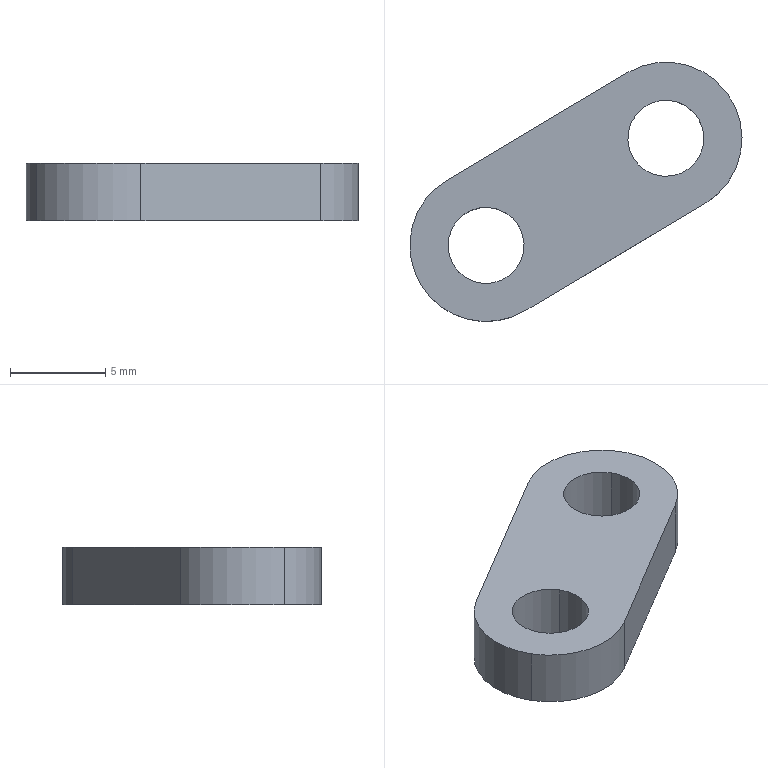Component | SolidWorks | JR-PL-JD-05ConnectingRod-2 | 1 solid | 11 faces | box 17.45 x 13.63 x 3 mm | volume 339 mm3 | cylinder 7 | plane 4 | commonest cylinder face diameters 4 x4 8 x3
build123d program:
from build123d import *

# Parameters (mm, degrees)
SKETCH1_R           = 2
BOSS_EXTRUDE1_DEPTH = 3


with BuildPart() as part:
    # Sketch1 → Boss-Extrude1 (new body)
    with BuildSketch(Plane.XY):
        with BuildLine():
            Line((0, 4), (11, 4))
            ThreePointArc((11, 4), (15, 0), (11, -4))
            Line((11, -4), (0, -4))
            ThreePointArc((0, -4), (-4, 0), (0, 4))
        make_face()
        Circle(SKETCH1_R, mode=Mode.SUBTRACT)
        with Locations((11, 0)):
            Circle(SKETCH1_R, mode=Mode.SUBTRACT)
    extrude(amount=BOSS_EXTRUDE1_DEPTH)


solid = part.part

# Placed as in the assembly
solid = solid.moved(Location((16.506, 30.452, 73.77), (0, 0, 30.78)))
STEP:
#1=COLOUR_RGB('',0.7922,0.8196,0.9333);
#2=FILL_AREA_STYLE_COLOUR('',#1);
#3=FILL_AREA_STYLE('',(#2));
#4=SURFACE_STYLE_FILL_AREA(#3);
#5=SURFACE_SIDE_STYLE('',(#4));
#6=SURFACE_STYLE_USAGE(.BOTH.,#5);
#7=PRESENTATION_STYLE_ASSIGNMENT((#6));
#8=CARTESIAN_POINT('',(0.9543,1.38,3.022));
#9=VERTEX_POINT('',#8);
#10=CARTESIAN_POINT('',(1.09,1.461,3.022));
#11=VERTEX_POINT('',#10);
#12=CARTESIAN_POINT('',(1.022,1.421,3.022));
#13=DIRECTION('',(0.,-0.,1.));
#14=DIRECTION('',(0.8591,0.5117,0.));
#15=AXIS2_PLACEMENT_3D('',#12,#13,#14);
#16=CIRCLE('',#15,0.07874);
#17=EDGE_CURVE('',#9,#11,#16,.T.);
#18=ORIENTED_EDGE('',*,*,#17,.T.);
#19=CARTESIAN_POINT('',(1.09,1.461,2.904));
#20=VERTEX_POINT('',#19);
#21=CARTESIAN_POINT('',(1.09,1.461,3.022));
#22=DIRECTION('',(-0.,0.,-1.));
#23=VECTOR('',#22,39.37);
#24=LINE('',#21,#23);
#25=EDGE_CURVE('',#11,#20,#24,.T.);
#26=ORIENTED_EDGE('',*,*,#25,.T.);
#27=CARTESIAN_POINT('',(0.9543,1.38,2.904));
#28=VERTEX_POINT('',#27);
#29=CARTESIAN_POINT('',(1.022,1.421,2.904));
#30=DIRECTION('',(0.,-0.,1.));
#31=DIRECTION('',(0.8591,0.5117,0.));
#32=AXIS2_PLACEMENT_3D('',#29,#30,#31);
#33=CIRCLE('',#32,0.07874);
#34=EDGE_CURVE('',#28,#20,#33,.T.);
#35=ORIENTED_EDGE('',*,*,#34,.F.);
#36=CARTESIAN_POINT('',(0.9543,1.38,3.022));
#37=DIRECTION('',(-0.,0.,-1.));
#38=VECTOR('',#37,39.37);
#39=LINE('',#36,#38);
#40=EDGE_CURVE('',#9,#28,#39,.T.);
#41=ORIENTED_EDGE('',*,*,#40,.F.);
#42=EDGE_LOOP('',(#18,#26,#35,#41));
#43=FACE_OUTER_BOUND('',#42,.T.);
#44=CARTESIAN_POINT('',(1.022,1.421,3.022));
#45=DIRECTION('',(-0.,0.,-1.));
#46=DIRECTION('',(-0.8591,-0.5117,0.));
#47=AXIS2_PLACEMENT_3D('',#44,#45,#46);
#48=CYLINDRICAL_SURFACE('',#47,0.07874);
#49=ADVANCED_FACE('',(#43),#48,.F.);
#50=CARTESIAN_POINT('',(0.5822,1.159,3.022));
#51=VERTEX_POINT('',#50);
#52=CARTESIAN_POINT('',(0.7175,1.239,3.022));
#53=VERTEX_POINT('',#52);
#54=CARTESIAN_POINT('',(0.6498,1.199,3.022));
#55=DIRECTION('',(0.,-0.,1.));
#56=DIRECTION('',(0.8591,0.5117,0.));
#57=AXIS2_PLACEMENT_3D('',#54,#55,#56);
#58=CIRCLE('',#57,0.07874);
#59=EDGE_CURVE('',#51,#53,#58,.T.);
#60=ORIENTED_EDGE('',*,*,#59,.T.);
#61=CARTESIAN_POINT('',(0.7175,1.239,2.904));
#62=VERTEX_POINT('',#61);
#63=CARTESIAN_POINT('',(0.7175,1.239,3.022));
#64=DIRECTION('',(-0.,0.,-1.));
#65=VECTOR('',#64,39.37);
#66=LINE('',#63,#65);
#67=EDGE_CURVE('',#53,#62,#66,.T.);
#68=ORIENTED_EDGE('',*,*,#67,.T.);
#69=CARTESIAN_POINT('',(0.5822,1.159,2.904));
#70=VERTEX_POINT('',#69);
#71=CARTESIAN_POINT('',(0.6498,1.199,2.904));
#72=DIRECTION('',(0.,-0.,1.));
#73=DIRECTION('',(0.8591,0.5117,0.));
#74=AXIS2_PLACEMENT_3D('',#71,#72,#73);
#75=CIRCLE('',#74,0.07874);
#76=EDGE_CURVE('',#70,#62,#75,.T.);
#77=ORIENTED_EDGE('',*,*,#76,.F.);
#78=CARTESIAN_POINT('',(0.5822,1.159,3.022));
#79=DIRECTION('',(-0.,0.,-1.));
#80=VECTOR('',#79,39.37);
#81=LINE('',#78,#80);
#82=EDGE_CURVE('',#51,#70,#81,.T.);
#83=ORIENTED_EDGE('',*,*,#82,.F.);
#84=EDGE_LOOP('',(#60,#68,#77,#83));
#85=FACE_OUTER_BOUND('',#84,.T.);
#86=CARTESIAN_POINT('',(0.6498,1.199,3.022));
#87=DIRECTION('',(-0.,0.,-1.));
#88=DIRECTION('',(-0.8591,-0.5117,0.));
#89=AXIS2_PLACEMENT_3D('',#86,#87,#88);
#90=CYLINDRICAL_SURFACE('',#89,0.07874);
#91=ADVANCED_FACE('',(#85),#90,.F.);
#92=CARTESIAN_POINT('',(0.5145,1.118,3.022));
#93=VERTEX_POINT('',#92);
#94=CARTESIAN_POINT('',(0.7304,1.064,3.022));
#95=VERTEX_POINT('',#94);
#96=CARTESIAN_POINT('',(0.6498,1.199,3.022));
#97=DIRECTION('',(0.,-0.,1.));
#98=DIRECTION('',(0.8591,0.5117,0.));
#99=AXIS2_PLACEMENT_3D('',#96,#97,#98);
#100=CIRCLE('',#99,0.1575);
#101=EDGE_CURVE('',#93,#95,#100,.T.);
#102=ORIENTED_EDGE('',*,*,#101,.F.);
#103=CARTESIAN_POINT('',(0.5145,1.118,2.904));
#104=VERTEX_POINT('',#103);
#105=CARTESIAN_POINT('',(0.5145,1.118,3.022));
#106=DIRECTION('',(-0.,0.,-1.));
#107=VECTOR('',#106,39.37);
#108=LINE('',#105,#107);
#109=EDGE_CURVE('',#93,#104,#108,.T.);
#110=ORIENTED_EDGE('',*,*,#109,.T.);
#111=CARTESIAN_POINT('',(0.7304,1.064,2.904));
#112=VERTEX_POINT('',#111);
#113=CARTESIAN_POINT('',(0.6498,1.199,2.904));
#114=DIRECTION('',(0.,-0.,1.));
#115=DIRECTION('',(0.8591,0.5117,0.));
#116=AXIS2_PLACEMENT_3D('',#113,#114,#115);
#117=CIRCLE('',#116,0.1575);
#118=EDGE_CURVE('',#104,#112,#117,.T.);
#119=ORIENTED_EDGE('',*,*,#118,.T.);
#120=CARTESIAN_POINT('',(0.7304,1.064,3.022));
#121=DIRECTION('',(-0.,0.,-1.));
#122=VECTOR('',#121,39.37);
#123=LINE('',#120,#122);
#124=EDGE_CURVE('',#95,#112,#123,.T.);
#125=ORIENTED_EDGE('',*,*,#124,.F.);
#126=EDGE_LOOP('',(#102,#110,#119,#125));
#127=FACE_OUTER_BOUND('',#126,.T.);
#128=CARTESIAN_POINT('',(0.6498,1.199,3.022));
#129=DIRECTION('',(-0.,0.,-1.));
#130=DIRECTION('',(-0.8591,-0.5117,0.));
#131=AXIS2_PLACEMENT_3D('',#128,#129,#130);
#132=CYLINDRICAL_SURFACE('',#131,0.1575);
#133=ADVANCED_FACE('',(#127),#132,.T.);
#134=ORIENTED_EDGE('',*,*,#59,.F.);
#135=CARTESIAN_POINT('',(0.6498,1.199,3.022));
#136=DIRECTION('',(0.,-0.,1.));
#137=DIRECTION('',(0.8591,0.5117,0.));
#138=AXIS2_PLACEMENT_3D('',#135,#136,#137);
#139=CIRCLE('',#138,0.07874);
#140=EDGE_CURVE('',#53,#51,#139,.T.);
#141=ORIENTED_EDGE('',*,*,#140,.F.);
#142=EDGE_LOOP('',(#134,#141));
#143=FACE_BOUND('',#142,.T.);
#144=CARTESIAN_POINT('',(0.5693,1.334,3.022));
#145=VERTEX_POINT('',#144);
#146=CARTESIAN_POINT('',(0.6498,1.199,3.022));
#147=DIRECTION('',(0.,-0.,1.));
#148=DIRECTION('',(0.8591,0.5117,0.));
#149=AXIS2_PLACEMENT_3D('',#146,#147,#148);
#150=CIRCLE('',#149,0.1575);
#151=EDGE_CURVE('',#145,#93,#150,.T.);
#152=ORIENTED_EDGE('',*,*,#151,.T.);
#153=ORIENTED_EDGE('',*,*,#101,.T.);
#154=CARTESIAN_POINT('',(1.102,1.285,3.022));
#155=VERTEX_POINT('',#154);
#156=CARTESIAN_POINT('',(0.7304,1.064,3.022));
#157=DIRECTION('',(0.8591,0.5117,-0.));
#158=VECTOR('',#157,39.37);
#159=LINE('',#156,#158);
#160=EDGE_CURVE('',#95,#155,#159,.T.);
#161=ORIENTED_EDGE('',*,*,#160,.T.);
#162=CARTESIAN_POINT('',(0.9413,1.556,3.022));
#163=VERTEX_POINT('',#162);
#164=CARTESIAN_POINT('',(1.022,1.421,3.022));
#165=DIRECTION('',(0.,-0.,1.));
#166=DIRECTION('',(0.8591,0.5117,0.));
#167=AXIS2_PLACEMENT_3D('',#164,#165,#166);
#168=CIRCLE('',#167,0.1575);
#169=EDGE_CURVE('',#155,#163,#168,.T.);
#170=ORIENTED_EDGE('',*,*,#169,.T.);
#171=CARTESIAN_POINT('',(0.5693,1.334,3.022));
#172=DIRECTION('',(-0.8591,-0.5117,0.));
#173=VECTOR('',#172,39.37);
#174=LINE('',#171,#173);
#175=EDGE_CURVE('',#163,#145,#174,.T.);
#176=ORIENTED_EDGE('',*,*,#175,.T.);
#177=EDGE_LOOP('',(#152,#153,#161,#170,#176));
#178=FACE_OUTER_BOUND('',#177,.T.);
#179=ORIENTED_EDGE('',*,*,#17,.F.);
#180=CARTESIAN_POINT('',(1.022,1.421,3.022));
#181=DIRECTION('',(0.,-0.,1.));
#182=DIRECTION('',(0.8591,0.5117,0.));
#183=AXIS2_PLACEMENT_3D('',#180,#181,#182);
#184=CIRCLE('',#183,0.07874);
#185=EDGE_CURVE('',#11,#9,#184,.T.);
#186=ORIENTED_EDGE('',*,*,#185,.F.);
#187=EDGE_LOOP('',(#179,#186));
#188=FACE_BOUND('',#187,.T.);
#189=CARTESIAN_POINT('',(0.6498,1.199,3.022));
#190=DIRECTION('',(0.,-0.,1.));
#191=DIRECTION('',(0.8591,0.5117,-0.));
#192=AXIS2_PLACEMENT_3D('',#189,#190,#191);
#193=PLANE('',#192);
#194=ADVANCED_FACE('',(#143,#178,#188),#193,.T.);
#195=CARTESIAN_POINT('',(0.5693,1.334,2.904));
#196=VERTEX_POINT('',#195);
#197=CARTESIAN_POINT('',(0.6498,1.199,2.904));
#198=DIRECTION('',(0.,-0.,1.));
#199=DIRECTION('',(0.8591,0.5117,0.));
#200=AXIS2_PLACEMENT_3D('',#197,#198,#199);
#201=CIRCLE('',#200,0.1575);
#202=EDGE_CURVE('',#196,#104,#201,.T.);
#203=ORIENTED_EDGE('',*,*,#202,.F.);
#204=CARTESIAN_POINT('',(0.9413,1.556,2.904));
#205=VERTEX_POINT('',#204);
#206=CARTESIAN_POINT('',(0.5693,1.334,2.904));
#207=DIRECTION('',(-0.8591,-0.5117,0.));
#208=VECTOR('',#207,39.37);
#209=LINE('',#206,#208);
#210=EDGE_CURVE('',#205,#196,#209,.T.);
#211=ORIENTED_EDGE('',*,*,#210,.F.);
#212=CARTESIAN_POINT('',(1.102,1.285,2.904));
#213=VERTEX_POINT('',#212);
#214=CARTESIAN_POINT('',(1.022,1.421,2.904));
#215=DIRECTION('',(0.,-0.,1.));
#216=DIRECTION('',(0.8591,0.5117,0.));
#217=AXIS2_PLACEMENT_3D('',#214,#215,#216);
#218=CIRCLE('',#217,0.1575);
#219=EDGE_CURVE('',#213,#205,#218,.T.);
#220=ORIENTED_EDGE('',*,*,#219,.F.);
#221=CARTESIAN_POINT('',(0.7304,1.064,2.904));
#222=DIRECTION('',(0.8591,0.5117,-0.));
#223=VECTOR('',#222,39.37);
#224=LINE('',#221,#223);
#225=EDGE_CURVE('',#112,#213,#224,.T.);
#226=ORIENTED_EDGE('',*,*,#225,.F.);
#227=ORIENTED_EDGE('',*,*,#118,.F.);
#228=EDGE_LOOP('',(#203,#211,#220,#226,#227));
#229=FACE_OUTER_BOUND('',#228,.T.);
#230=ORIENTED_EDGE('',*,*,#76,.T.);
#231=CARTESIAN_POINT('',(0.6498,1.199,2.904));
#232=DIRECTION('',(0.,-0.,1.));
#233=DIRECTION('',(0.8591,0.5117,0.));
#234=AXIS2_PLACEMENT_3D('',#231,#232,#233);
#235=CIRCLE('',#234,0.07874);
#236=EDGE_CURVE('',#62,#70,#235,.T.);
#237=ORIENTED_EDGE('',*,*,#236,.T.);
#238=EDGE_LOOP('',(#230,#237));
#239=FACE_BOUND('',#238,.T.);
#240=ORIENTED_EDGE('',*,*,#34,.T.);
#241=CARTESIAN_POINT('',(1.022,1.421,2.904));
#242=DIRECTION('',(0.,-0.,1.));
#243=DIRECTION('',(0.8591,0.5117,0.));
#244=AXIS2_PLACEMENT_3D('',#241,#242,#243);
#245=CIRCLE('',#244,0.07874);
#246=EDGE_CURVE('',#20,#28,#245,.T.);
#247=ORIENTED_EDGE('',*,*,#246,.T.);
#248=EDGE_LOOP('',(#240,#247));
#249=FACE_BOUND('',#248,.T.);
#250=CARTESIAN_POINT('',(0.6498,1.199,2.904));
#251=DIRECTION('',(0.,-0.,1.));
#252=DIRECTION('',(0.8591,0.5117,-0.));
#253=AXIS2_PLACEMENT_3D('',#250,#251,#252);
#254=PLANE('',#253);
#255=ADVANCED_FACE('',(#229,#239,#249),#254,.F.);
#256=ORIENTED_EDGE('',*,*,#109,.F.);
#257=ORIENTED_EDGE('',*,*,#151,.F.);
#258=CARTESIAN_POINT('',(0.5693,1.334,3.022));
#259=DIRECTION('',(-0.,0.,-1.));
#260=VECTOR('',#259,39.37);
#261=LINE('',#258,#260);
#262=EDGE_CURVE('',#145,#196,#261,.T.);
#263=ORIENTED_EDGE('',*,*,#262,.T.);
#264=ORIENTED_EDGE('',*,*,#202,.T.);
#265=EDGE_LOOP('',(#256,#257,#263,#264));
#266=FACE_OUTER_BOUND('',#265,.T.);
#267=CARTESIAN_POINT('',(0.6498,1.199,3.022));
#268=DIRECTION('',(-0.,0.,-1.));
#269=DIRECTION('',(-0.8591,-0.5117,0.));
#270=AXIS2_PLACEMENT_3D('',#267,#268,#269);
#271=CYLINDRICAL_SURFACE('',#270,0.1575);
#272=ADVANCED_FACE('',(#266),#271,.T.);
#273=ORIENTED_EDGE('',*,*,#225,.T.);
#274=CARTESIAN_POINT('',(1.102,1.285,3.022));
#275=DIRECTION('',(-0.,0.,-1.));
#276=VECTOR('',#275,39.37);
#277=LINE('',#274,#276);
#278=EDGE_CURVE('',#155,#213,#277,.T.);
#279=ORIENTED_EDGE('',*,*,#278,.F.);
#280=ORIENTED_EDGE('',*,*,#160,.F.);
#281=ORIENTED_EDGE('',*,*,#124,.T.);
#282=EDGE_LOOP('',(#273,#279,#280,#281));
#283=FACE_OUTER_BOUND('',#282,.T.);
#284=CARTESIAN_POINT('',(0.7304,1.064,3.022));
#285=DIRECTION('',(-0.5117,0.8591,0.));
#286=DIRECTION('',(0.,-0.,1.));
#287=AXIS2_PLACEMENT_3D('',#284,#285,#286);
#288=PLANE('',#287);
#289=ADVANCED_FACE('',(#283),#288,.F.);
#290=ORIENTED_EDGE('',*,*,#219,.T.);
#291=CARTESIAN_POINT('',(0.9413,1.556,3.022));
#292=DIRECTION('',(-0.,0.,-1.));
#293=VECTOR('',#292,39.37);
#294=LINE('',#291,#293);
#295=EDGE_CURVE('',#163,#205,#294,.T.);
#296=ORIENTED_EDGE('',*,*,#295,.F.);
#297=ORIENTED_EDGE('',*,*,#169,.F.);
#298=ORIENTED_EDGE('',*,*,#278,.T.);
#299=EDGE_LOOP('',(#290,#296,#297,#298));
#300=FACE_OUTER_BOUND('',#299,.T.);
#301=CARTESIAN_POINT('',(1.022,1.421,3.022));
#302=DIRECTION('',(-0.,0.,-1.));
#303=DIRECTION('',(-0.8591,-0.5117,0.));
#304=AXIS2_PLACEMENT_3D('',#301,#302,#303);
#305=CYLINDRICAL_SURFACE('',#304,0.1575);
#306=ADVANCED_FACE('',(#300),#305,.T.);
#307=ORIENTED_EDGE('',*,*,#210,.T.);
#308=ORIENTED_EDGE('',*,*,#262,.F.);
#309=ORIENTED_EDGE('',*,*,#175,.F.);
#310=ORIENTED_EDGE('',*,*,#295,.T.);
#311=EDGE_LOOP('',(#307,#308,#309,#310));
#312=FACE_OUTER_BOUND('',#311,.T.);
#313=CARTESIAN_POINT('',(0.5693,1.334,3.022));
#314=DIRECTION('',(0.5117,-0.8591,-0.));
#315=DIRECTION('',(-0.,0.,-1.));
#316=AXIS2_PLACEMENT_3D('',#313,#314,#315);
#317=PLANE('',#316);
#318=ADVANCED_FACE('',(#312),#317,.F.);
#319=ORIENTED_EDGE('',*,*,#67,.F.);
#320=ORIENTED_EDGE('',*,*,#140,.T.);
#321=ORIENTED_EDGE('',*,*,#82,.T.);
#322=ORIENTED_EDGE('',*,*,#236,.F.);
#323=EDGE_LOOP('',(#319,#320,#321,#322));
#324=FACE_OUTER_BOUND('',#323,.T.);
#325=CARTESIAN_POINT('',(0.6498,1.199,3.022));
#326=DIRECTION('',(-0.,0.,-1.));
#327=DIRECTION('',(-0.8591,-0.5117,0.));
#328=AXIS2_PLACEMENT_3D('',#325,#326,#327);
#329=CYLINDRICAL_SURFACE('',#328,0.07874);
#330=ADVANCED_FACE('',(#324),#329,.F.);
#331=ORIENTED_EDGE('',*,*,#25,.F.);
#332=ORIENTED_EDGE('',*,*,#185,.T.);
#333=ORIENTED_EDGE('',*,*,#40,.T.);
#334=ORIENTED_EDGE('',*,*,#246,.F.);
#335=EDGE_LOOP('',(#331,#332,#333,#334));
#336=FACE_OUTER_BOUND('',#335,.T.);
#337=CARTESIAN_POINT('',(1.022,1.421,3.022));
#338=DIRECTION('',(-0.,0.,-1.));
#339=DIRECTION('',(-0.8591,-0.5117,0.));
#340=AXIS2_PLACEMENT_3D('',#337,#338,#339);
#341=CYLINDRICAL_SURFACE('',#340,0.07874);
#342=ADVANCED_FACE('',(#336),#341,.F.);
#343=CLOSED_SHELL('',(#49,#91,#133,#194,#255,#272,#289,#306,#318,#330,#342));
#344=MANIFOLD_SOLID_BREP('',#343);
#345=STYLED_ITEM('',(#7),#344);
#346=PRESENTATION_LAYER_ASSIGNMENT('','',(#345));
#347=CARTESIAN_POINT('',(0.,0.,0.));
#348=DIRECTION('',(0.,0.,1.));
#349=DIRECTION('',(1.,0.,0.));
#350=AXIS2_PLACEMENT_3D('',#347,#348,#349);
#351=(LENGTH_UNIT()NAMED_UNIT(*)SI_UNIT($,.METRE.));
#352=LENGTH_MEASURE_WITH_UNIT(LENGTH_MEASURE(0.0254),#351);
#353=DIMENSIONAL_EXPONENTS(1.,0.,0.,0.,0.,0.,0.);
#354=(CONVERSION_BASED_UNIT('',#352)LENGTH_UNIT()NAMED_UNIT(#353));
#355=UNCERTAINTY_MEASURE_WITH_UNIT(LENGTH_MEASURE(0.00001),#354,'','');
#356=(NAMED_UNIT(*)PLANE_ANGLE_UNIT()SI_UNIT($,.RADIAN.));
#357=(NAMED_UNIT(*)SI_UNIT($,.STERADIAN.)SOLID_ANGLE_UNIT());
#358=(GEOMETRIC_REPRESENTATION_CONTEXT(3)GLOBAL_UNCERTAINTY_ASSIGNED_CONTEXT((#355))GLOBAL_UNIT_ASSIGNED_CONTEXT((#354,#356,#357))REPRESENTATION_CONTEXT('',''));
#359=ADVANCED_BREP_SHAPE_REPRESENTATION('',(#344,#350),#358);
#360=(LENGTH_UNIT()NAMED_UNIT(*)SI_UNIT($,.METRE.));
#361=LENGTH_MEASURE_WITH_UNIT(LENGTH_MEASURE(0.0254),#360);
#362=DIMENSIONAL_EXPONENTS(1.,0.,0.,0.,0.,0.,0.);
#363=(CONVERSION_BASED_UNIT('',#361)LENGTH_UNIT()NAMED_UNIT(#362));
#364=UNCERTAINTY_MEASURE_WITH_UNIT(LENGTH_MEASURE(0.00001),#363,'','');
#365=(NAMED_UNIT(*)PLANE_ANGLE_UNIT()SI_UNIT($,.RADIAN.));
#366=(NAMED_UNIT(*)SI_UNIT($,.STERADIAN.)SOLID_ANGLE_UNIT());
#367=(GEOMETRIC_REPRESENTATION_CONTEXT(3)GLOBAL_UNCERTAINTY_ASSIGNED_CONTEXT((#364))GLOBAL_UNIT_ASSIGNED_CONTEXT((#363,#365,#366))REPRESENTATION_CONTEXT('',''));
#368=MECHANICAL_DESIGN_GEOMETRIC_PRESENTATION_REPRESENTATION('',(#345),#367);